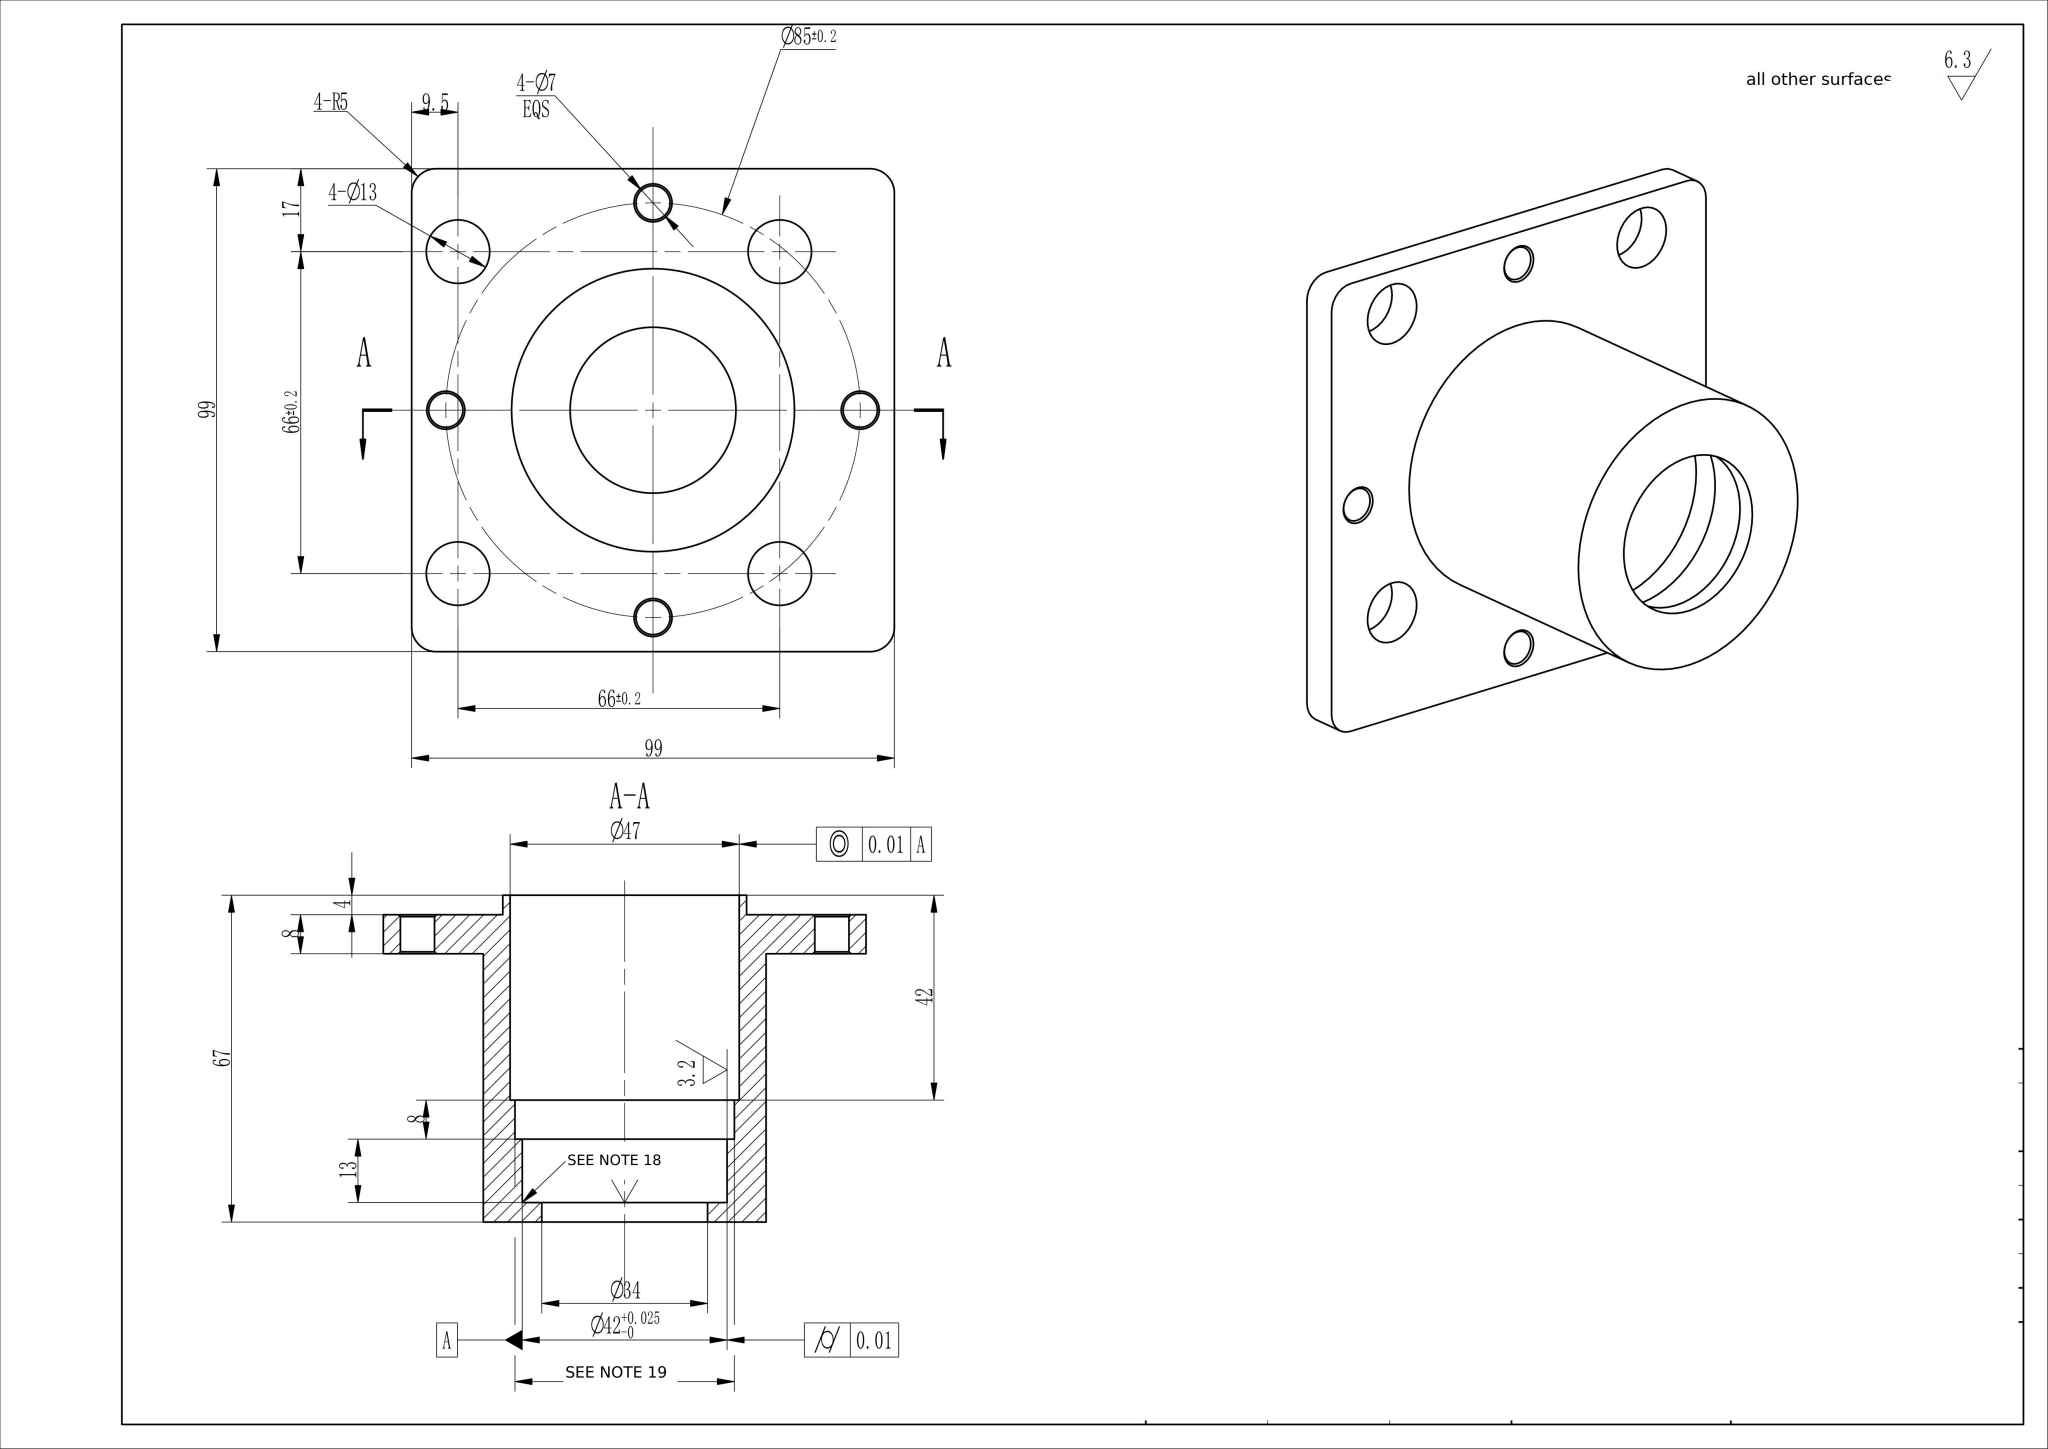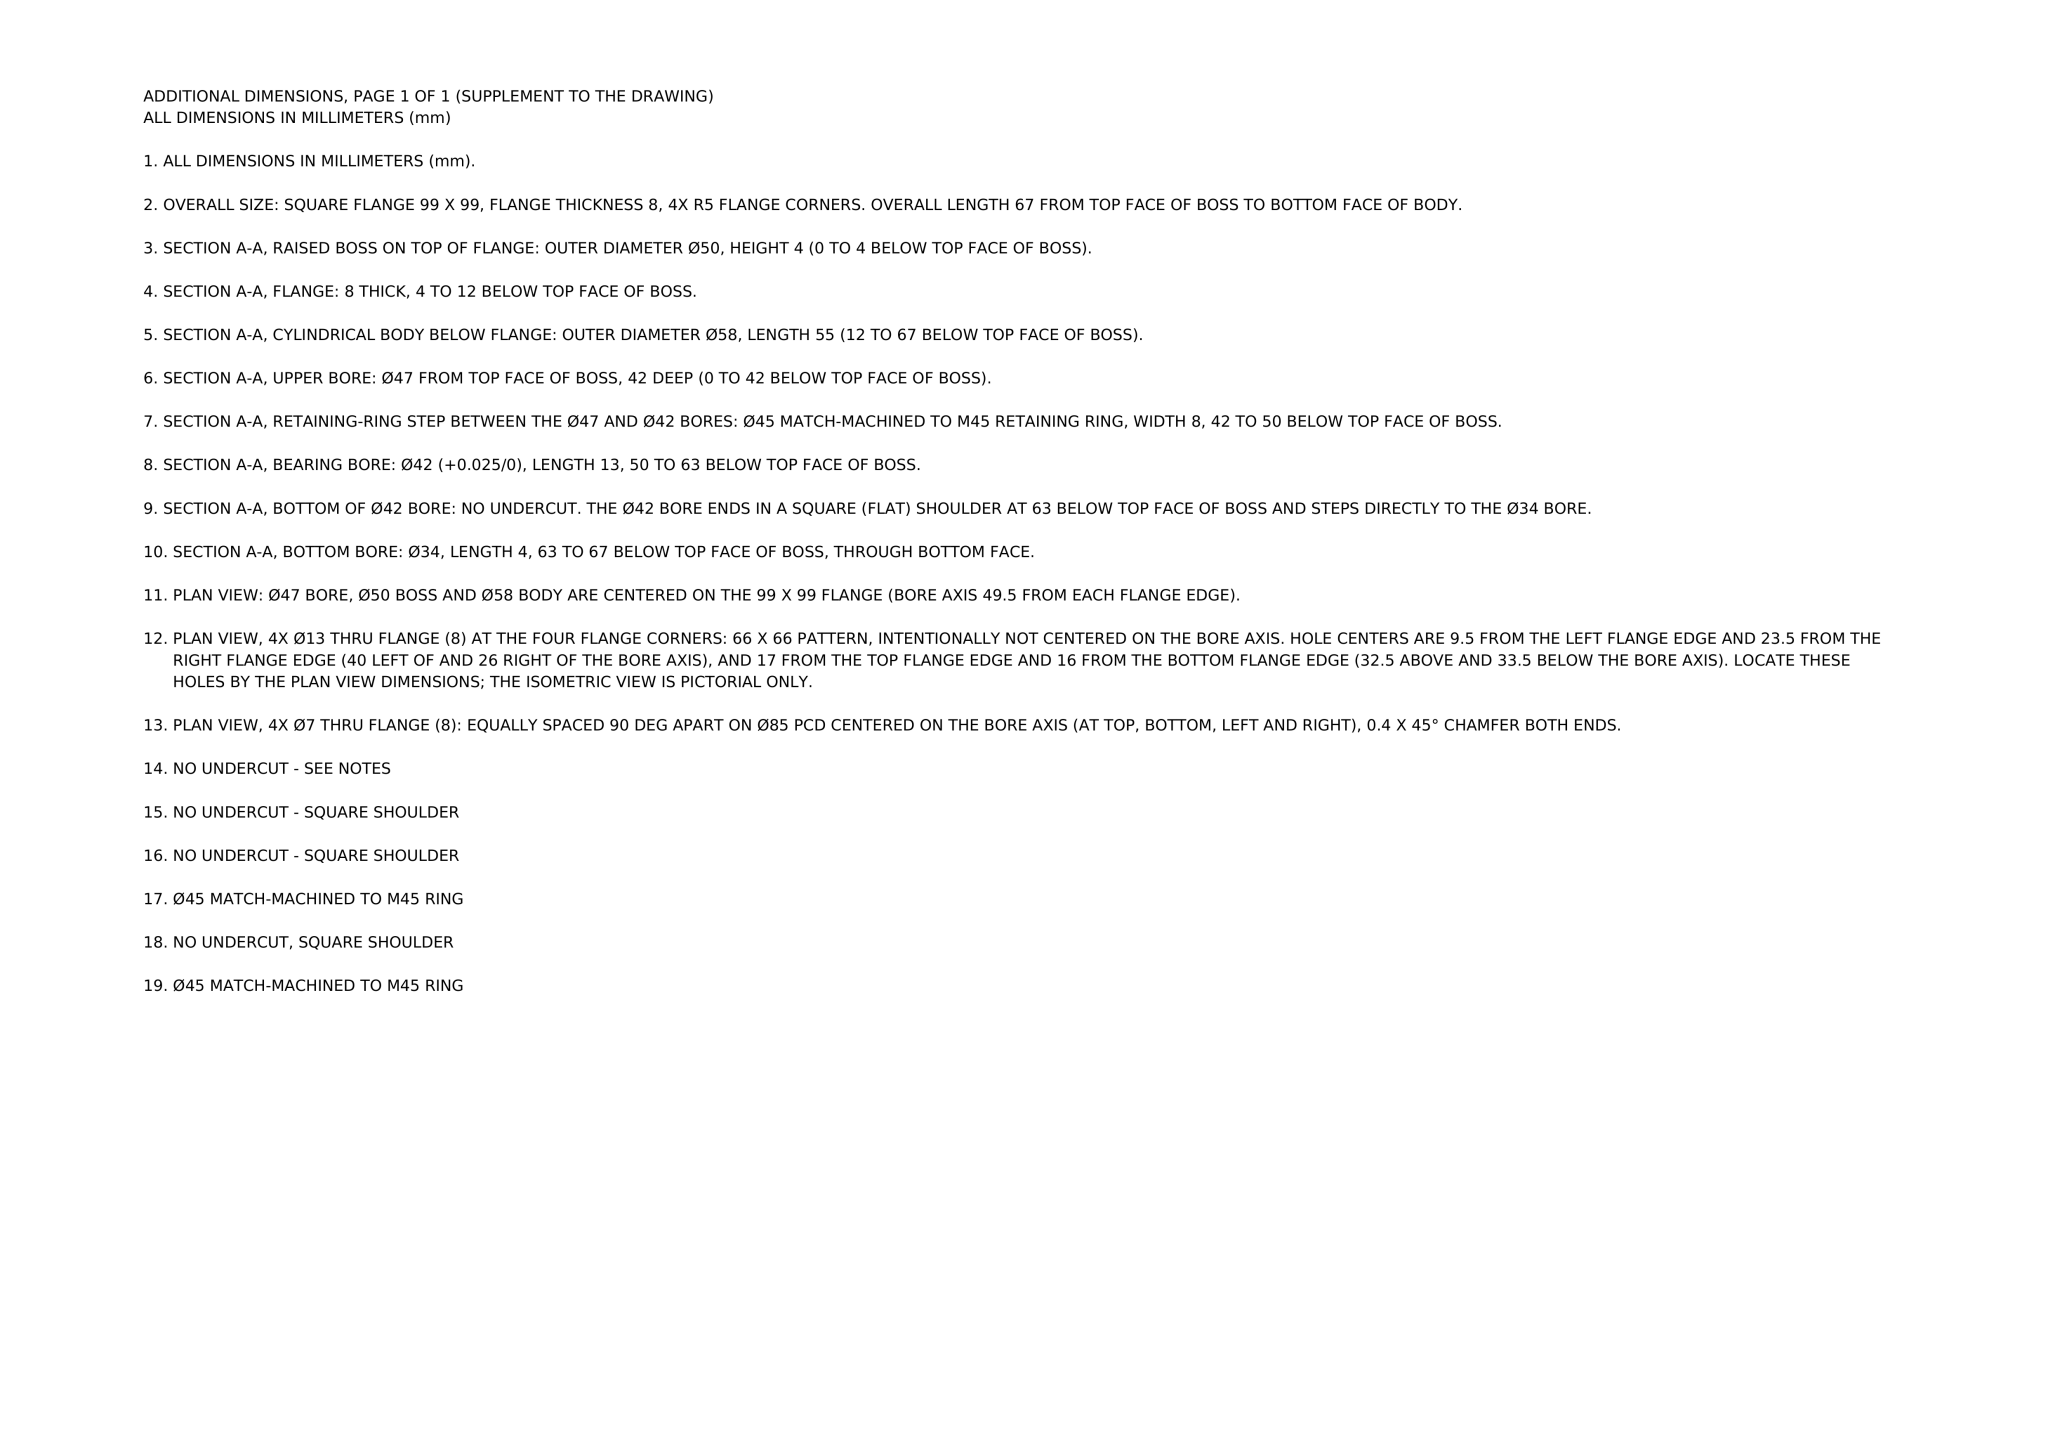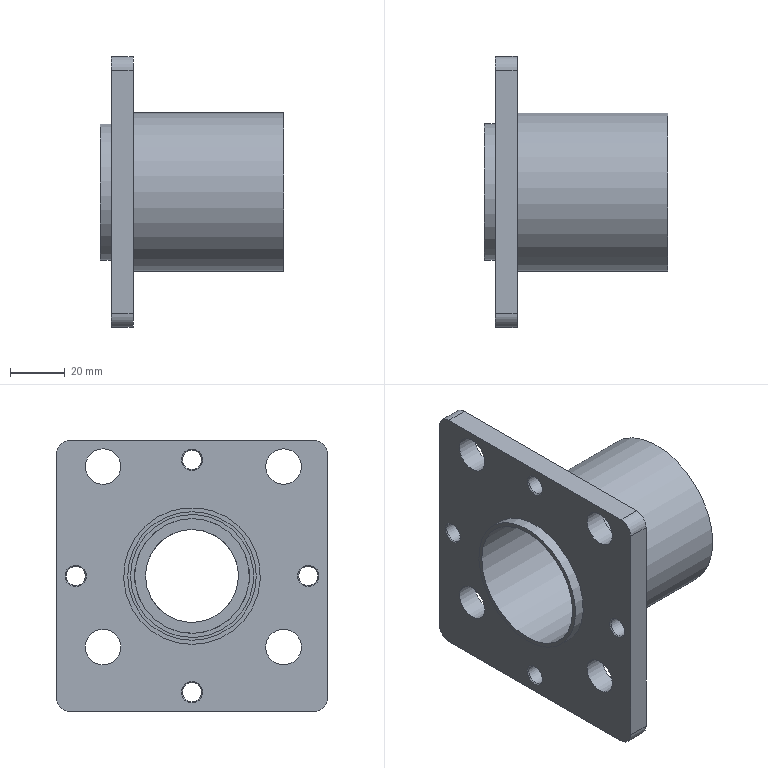Part | NX | mm | 1 solid | 37 faces | box 67 x 99 x 99 mm | volume 118678 mm3 | cylinder 18 | plane 11 | cone 8 | commonest cylinder face diameters 10 x4 13 x4 7 x4 58 x1 47 x1 45 x1 42 x1 34 x1